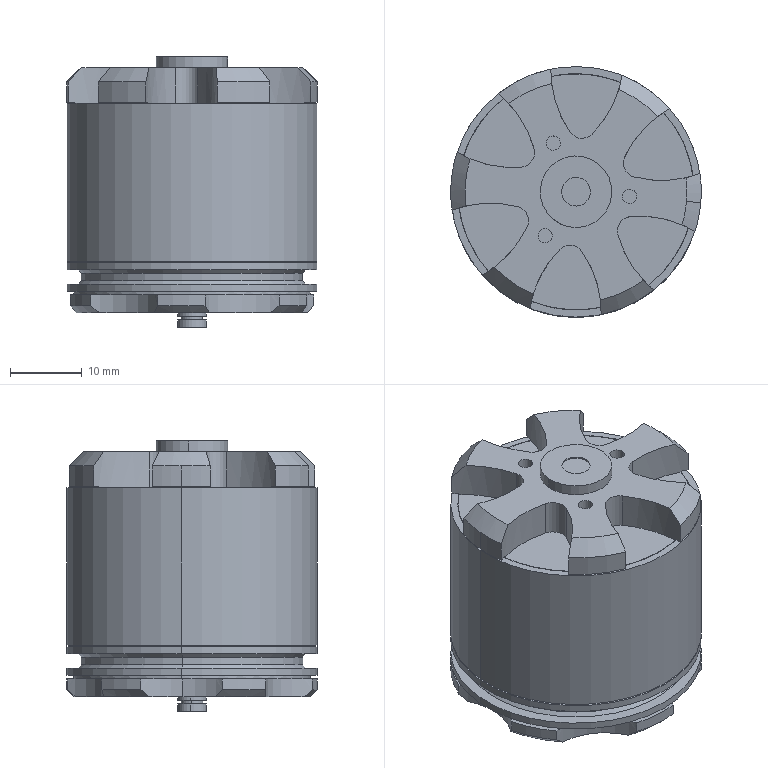Component | SolidWorks | Motor-2 | 1 solid | 175 faces | box 35 x 35 x 37.75 mm | volume 28973 mm3 | cylinder 106 | plane 44 | cone 25 | commonest cylinder face diameters 4 x26 35 x19 2.5 x16 30 x12 18 x7 2 x6 33 x4 16 x4
build123d program:
from build123d import *

# Parameters (mm, degrees)
CUT_EXTRUDE1_DEPTH             = 5
CIRPATTERN1_COUNT              = 6
SKETCH3_R                      = 1
CUT_EXTRUDE2_DEPTH             = 7
CUT_EXTRUDE3_DEPTH             = 5
CIRPATTERN2_COUNT              = 4
CUT_EXTRUDE4_REACH             = 45.481
SKETCH5_R                      = 9
CIRPATTERN3_COUNT              = 6
F_2_5_2_5_DIAMETER_HOLE1_D     = 2.5
F_2_5_2_5_DIAMETER_HOLE1_DEPTH = 8.5
F_2_5_2_5_DIAMETER_HOLE1_TIP   = 0.7511


with BuildPart() as part:
    # Sketch1 → Revolve1 (revolve)
    with BuildSketch(Plane.XY, mode=Mode.PRIVATE) as revolve1_sk:
        Polygon((0, 0), (-2, 0), (-2, 1), (-1.5, 1), (-1.5, 1.5), (-2, 1.5), (-2, 2), (-16.5, 2), (-17.5, 3), (-17.5, 4.5), (-16.5, 4.5), (-16.5, 5), (-17.5, 5), (-17.5, 6), (-16, 6), (-15.5, 6.5), (-15.5, 7.5), (-16, 8), (-17.5, 8), (-17.5, 9), (-7.5, 9), (-7.5, 9.2), (-17.5, 9.2), (-17.5, 31.2), (-16.5, 31.2), (-16.5, 31.4), (-17.5, 31.4), (-17.5, 34.25), (-15.5, 36.25), (-5, 36.25), (-5, 37.75), (-2, 37.75), (-2, 37.55), (0, 37.55), align=None)
    revolve(revolve1_sk.sketch.rotate(Axis((0, 37.55, 0), (0, -1, 0)), 270), axis=Axis((0, 37.55, 0), (0, -1, 0)))

    # Sketch2 → Cut-Extrude1 (cut)
    with BuildSketch(Plane(origin=(0, 36.25, 0), x_dir=(1, 0, 0), z_dir=(0, 1, 0))):
        with BuildLine():
            ThreePointArc((-8.215, -1.532), (-7.5, 0), (-8.215, 1.532))
            ThreePointArc((-8.215, 1.532), (-12.219, 3.941), (-16.771, 5))
            ThreePointArc((-16.771, 5), (-17.5, 0), (-16.771, -5))
            ThreePointArc((-16.771, -5), (-12.219, -3.941), (-8.215, -1.532))
        make_face()
    cut_extrude1 = extrude(amount=-CUT_EXTRUDE1_DEPTH, mode=Mode.SUBTRACT)

    # CirPattern1: Cut-Extrude1 ×6 about axis
    cirpattern1_axis = Axis((0, 0, 0), (0, 1, 0))
    for i in range(1, CIRPATTERN1_COUNT):
        add(cut_extrude1.rotate(cirpattern1_axis, i * 360 / CIRPATTERN1_COUNT), mode=Mode.SUBTRACT)

    # Sketch3 → Cut-Extrude2 (cut)
    with BuildSketch(Plane(origin=(0, 36.25, 0), x_dir=(1, 0, 0), z_dir=(0, 1, 0))):
        with Locations(Location((0, 7.5, 0), (0, 0, 270))):
            Circle(SKETCH3_R)
        with Locations(Location((-6.495, -3.75, 0), (0, 0, 270))):
            Circle(SKETCH3_R)
        with Locations(Location((6.495, -3.75, 0), (0, 0, 270))):
            Circle(SKETCH3_R)
    extrude(amount=-CUT_EXTRUDE2_DEPTH, mode=Mode.SUBTRACT)

    # Sketch4 → Cut-Extrude3 (cut)
    with BuildSketch(Plane.XZ.offset(-2)):
        with BuildLine():
            ThreePointArc((10.392, 6), (8.485, 8.485), (6, 10.392))
            ThreePointArc((6, 10.392), (3.268, 9.66), (4, 6.928))
            ThreePointArc((4, 6.928), (5.657, 5.657), (6.928, 4))
            ThreePointArc((6.928, 4), (9.66, 3.268), (10.392, 6))
        make_face()
    cut_extrude3 = extrude(amount=-CUT_EXTRUDE3_DEPTH, mode=Mode.SUBTRACT)

    # CirPattern2: Cut-Extrude3 ×4 about axis
    cirpattern2_axis = Axis((0, 0, 0), (0, 1, 0))
    for i in range(1, CIRPATTERN2_COUNT):
        add(cut_extrude3.rotate(cirpattern2_axis, i * 360 / CIRPATTERN2_COUNT), mode=Mode.SUBTRACT)

    # Cut-Extrude4: up to this face of the body (flat: up to its plane)
    cut_extrude4_end = Plane(part.part.faces().sort_by_distance((0, 4.5, -17.005))[0])
    # Sketch5 → Cut-Extrude4 (cut, up to the picked face)
    with BuildSketch(Plane.XZ.offset(-2), mode=Mode.PRIVATE) as cut_extrude4_sk1:
        with Locations((0, 23.5)):
            Circle(SKETCH5_R)
    cut_extrude4_tool1 = split(extrude(cut_extrude4_sk1.sketch, amount=-CUT_EXTRUDE4_REACH, mode=Mode.PRIVATE), bisect_by=cut_extrude4_end, keep=Keep.BOTH, mode=Mode.PRIVATE)
    cut_extrude4 = cut_extrude4_tool1.solids().sort_by(Axis((0, 2, 23.5), (0, 1, 0)))[0]
    add(cut_extrude4, mode=Mode.SUBTRACT)

    # CirPattern3: Cut-Extrude4 ×6 about axis
    cirpattern3_axis = Axis((0, 0, 0), (0, 1, 0))
    for i in range(1, CIRPATTERN3_COUNT):
        add(cut_extrude4.rotate(cirpattern3_axis, i * 360 / CIRPATTERN3_COUNT), mode=Mode.SUBTRACT)

    # 2.5 _2.5_ Diameter Hole1
    with Locations(Plane(origin=(0, 2, 12.5), x_dir=(0, 0, -1), z_dir=(0, -1, 0))):
        with Locations((0, 0), (12.5, 9.5), (25, 0), (12.5, -9.5)):
            Hole(F_2_5_2_5_DIAMETER_HOLE1_D / 2, depth=F_2_5_2_5_DIAMETER_HOLE1_DEPTH)
            with Locations((0, 0, -(F_2_5_2_5_DIAMETER_HOLE1_DEPTH + F_2_5_2_5_DIAMETER_HOLE1_TIP / 2))):  # 118° drill point
                Cone(0, F_2_5_2_5_DIAMETER_HOLE1_D / 2, F_2_5_2_5_DIAMETER_HOLE1_TIP, mode=Mode.SUBTRACT)


solid = part.part

# Placed as in the assembly
solid = solid.moved(Location((-179.217, -162.42, 1040.6), (-90, -85, -180)))